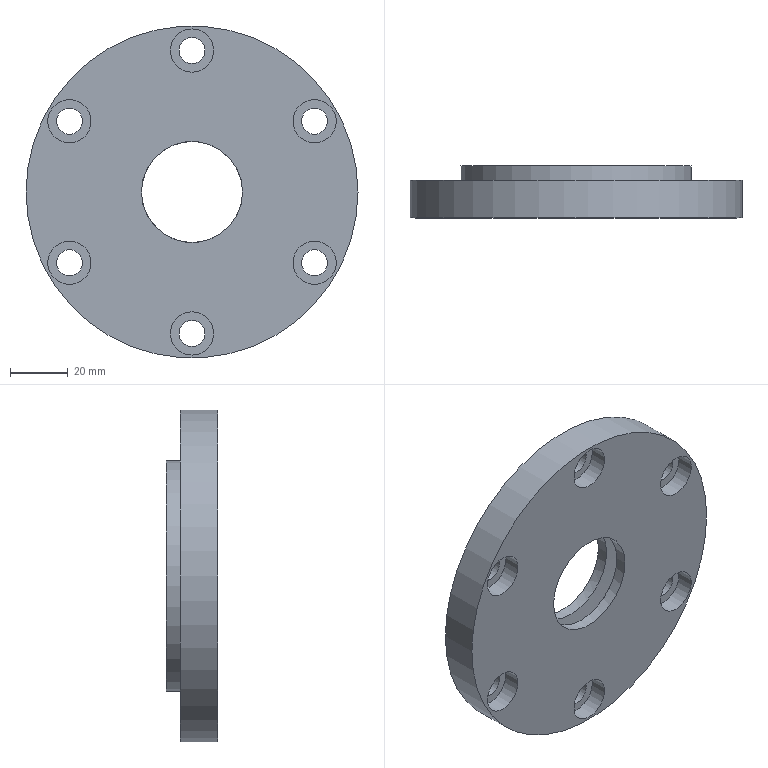Component | NX | END_CAP_2 | 1 solid | 30 faces | volume 116671 mm3 | cylinder 18 | plane 10 | cone 2 | commonest cylinder face diameters 9 x6 15 x6 35 x2 80 x1 68 x1 115 x1 48 x1